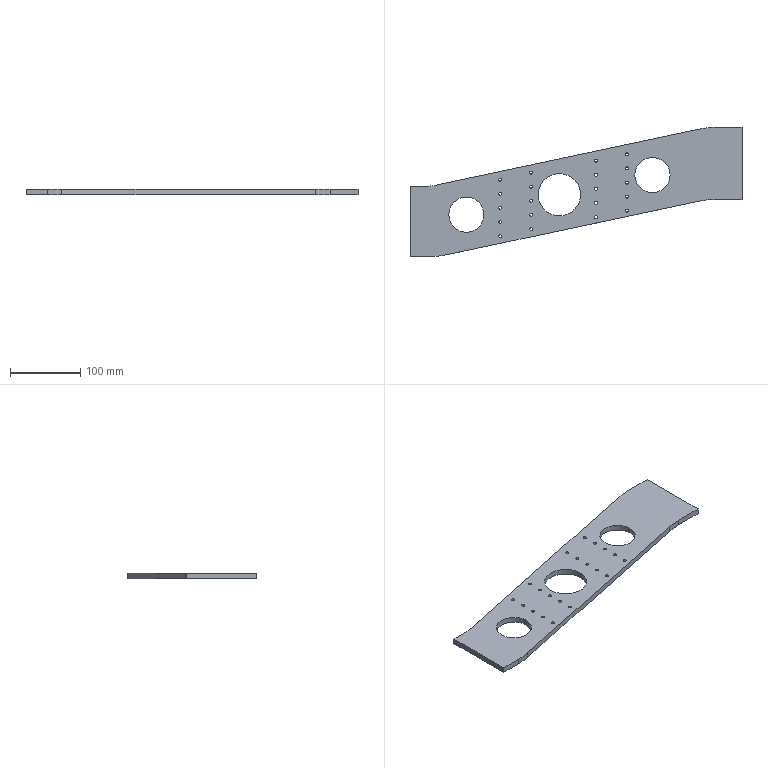Component | SolidWorks | 1VibrationTrackGuidePlate9.26-2 | 1 solid | 60 faces | volume 328522 mm3 | cylinder 50 | plane 10 | commonest cylinder face diameters 4.2 x40 50 x4 200 x3 60 x2 80 x1